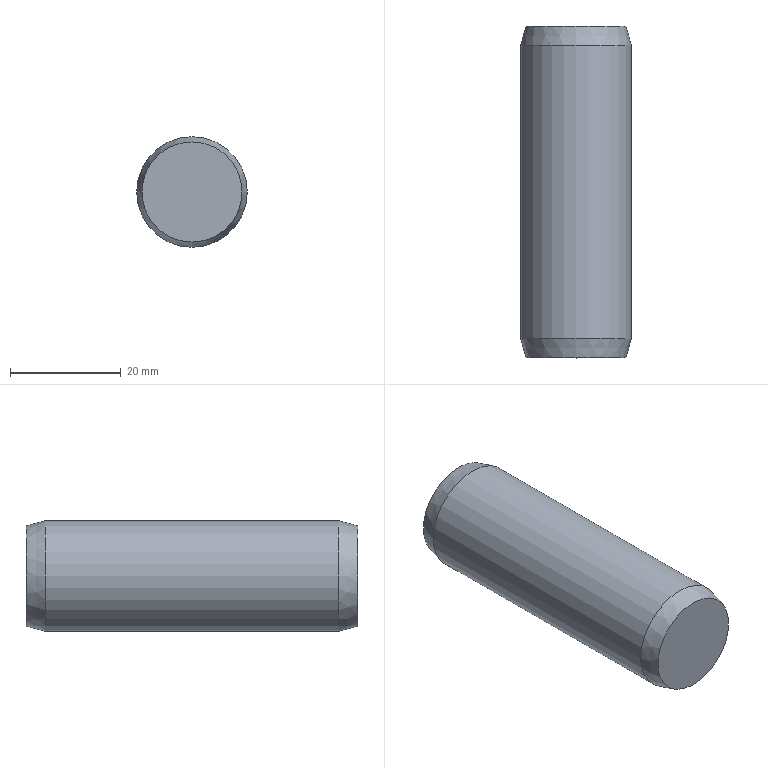Component | NX | GB-T119_1-2000_20X60 | 1 solid | 5 faces | box 20 x 60 x 20 mm | volume 18650 mm3 | plane 2 | cone 2 | cylinder 1 | commonest cylinder face diameters 20 x1
STEP:
#1=CARTESIAN_POINT('',(0.,0.,0.));
#2=DIRECTION('',(0.,0.,1.));
#3=DIRECTION('',(1.,0.,0.));
#4=AXIS2_PLACEMENT_3D('',#1,#2,#3);
#5=CARTESIAN_POINT('',(-170.,-110.,276.562));
#6=VERTEX_POINT('',#5);
#7=CARTESIAN_POINT('',(-170.,-110.,267.5));
#8=DIRECTION('',(0.,-1.,0.));
#9=DIRECTION('',(0.,0.,1.));
#10=AXIS2_PLACEMENT_3D('',#7,#8,#9);
#11=CIRCLE('',#10,9.062);
#12=CARTESIAN_POINT('',(-170.,-110.,267.5));
#13=DIRECTION('',(0.,-1.,0.));
#14=DIRECTION('',(0.,0.,1.));
#15=AXIS2_PLACEMENT_3D('',#12,#13,#14);
#16=PLANE('',#15);
#17=CARTESIAN_POINT('',(0.,0.));
#18=DIRECTION('',(1.,0.));
#19=AXIS2_PLACEMENT_2D('',#17,#18);
#20=CIRCLE('',#19,9.062);
#21=(GEOMETRIC_REPRESENTATION_CONTEXT(2)PARAMETRIC_REPRESENTATION_CONTEXT()REPRESENTATION_CONTEXT('',''));
#22=DEFINITIONAL_REPRESENTATION('',(#20),#21);
#23=PCURVE('',#16,#22);
#24=CARTESIAN_POINT('',(-170.,-110.,267.5));
#25=DIRECTION('',(0.,1.,0.));
#26=DIRECTION('',(0.,0.,-1.));
#27=AXIS2_PLACEMENT_3D('',#24,#25,#26);
#28=CONICAL_SURFACE('',#27,9.062,0.2618);
#29=CARTESIAN_POINT('',(9.425,-0.));
#30=DIRECTION('',(-1.,0.));
#31=VECTOR('',#30,1.);
#32=LINE('',#29,#31);
#33=(GEOMETRIC_REPRESENTATION_CONTEXT(2)PARAMETRIC_REPRESENTATION_CONTEXT()REPRESENTATION_CONTEXT('',''));
#34=DEFINITIONAL_REPRESENTATION('',(#32),#33);
#35=PCURVE('',#28,#34);
#36=SURFACE_CURVE('',#11,(#23,#35),.PCURVE_S1.);
#37=EDGE_CURVE('',#6,#6,#36,.T.);
#38=ORIENTED_EDGE('',*,*,#37,.T.);
#39=EDGE_LOOP('',(#38));
#40=FACE_BOUND('',#39,.T.);
#41=ADVANCED_FACE('',(#40),#16,.T.);
#42=CARTESIAN_POINT('',(-170.,-106.5,277.5));
#43=VERTEX_POINT('',#42);
#44=CARTESIAN_POINT('',(-170.,-106.5,267.5));
#45=DIRECTION('',(0.,-1.,0.));
#46=DIRECTION('',(0.,0.,1.));
#47=AXIS2_PLACEMENT_3D('',#44,#45,#46);
#48=CIRCLE('',#47,10.);
#49=CARTESIAN_POINT('',(9.425,3.5));
#50=DIRECTION('',(-1.,0.));
#51=VECTOR('',#50,1.);
#52=LINE('',#49,#51);
#53=(GEOMETRIC_REPRESENTATION_CONTEXT(2)PARAMETRIC_REPRESENTATION_CONTEXT()REPRESENTATION_CONTEXT('',''));
#54=DEFINITIONAL_REPRESENTATION('',(#52),#53);
#55=PCURVE('',#28,#54);
#56=CARTESIAN_POINT('',(-170.,-50.,267.5));
#57=DIRECTION('',(0.,-1.,0.));
#58=DIRECTION('',(0.,0.,1.));
#59=AXIS2_PLACEMENT_3D('',#56,#57,#58);
#60=CYLINDRICAL_SURFACE('',#59,10.);
#61=CARTESIAN_POINT('',(0.,56.5));
#62=DIRECTION('',(1.,0.));
#63=VECTOR('',#62,1.);
#64=LINE('',#61,#63);
#65=(GEOMETRIC_REPRESENTATION_CONTEXT(2)PARAMETRIC_REPRESENTATION_CONTEXT()REPRESENTATION_CONTEXT('',''));
#66=DEFINITIONAL_REPRESENTATION('',(#64),#65);
#67=PCURVE('',#60,#66);
#68=SURFACE_CURVE('',#48,(#55,#67),.PCURVE_S1.);
#69=EDGE_CURVE('',#43,#43,#68,.T.);
#70=ORIENTED_EDGE('',*,*,#69,.T.);
#71=CARTESIAN_POINT('',(-170.,-110.,276.562));
#72=CARTESIAN_POINT('',(-170.,-106.5,277.5));
#73=B_SPLINE_CURVE_WITH_KNOTS('',1,(#71,#72),.UNSPECIFIED.,.F.,.F.,(2,2),(-0.,3.623),.PIECEWISE_BEZIER_KNOTS.);
#74=CARTESIAN_POINT('',(3.142,0.));
#75=DIRECTION('',(0.,1.));
#76=VECTOR('',#75,1.);
#77=LINE('',#74,#76);
#78=(GEOMETRIC_REPRESENTATION_CONTEXT(2)PARAMETRIC_REPRESENTATION_CONTEXT()REPRESENTATION_CONTEXT('',''));
#79=DEFINITIONAL_REPRESENTATION('',(#77),#78);
#80=PCURVE('',#28,#79);
#81=CARTESIAN_POINT('',(9.425,0.));
#82=DIRECTION('',(0.,1.));
#83=VECTOR('',#82,1.);
#84=LINE('',#81,#83);
#85=(GEOMETRIC_REPRESENTATION_CONTEXT(2)PARAMETRIC_REPRESENTATION_CONTEXT()REPRESENTATION_CONTEXT('',''));
#86=DEFINITIONAL_REPRESENTATION('',(#84),#85);
#87=PCURVE('',#28,#86);
#88=SEAM_CURVE('',#73,(#80,#87),.PCURVE_S1.);
#89=EDGE_CURVE('',#6,#43,#88,.T.);
#90=ORIENTED_EDGE('',*,*,#89,.F.);
#91=ORIENTED_EDGE('',*,*,#37,.F.);
#92=ORIENTED_EDGE('',*,*,#89,.T.);
#93=EDGE_LOOP('',(#70,#90,#91,#92));
#94=FACE_BOUND('',#93,.T.);
#95=ADVANCED_FACE('',(#94),#28,.T.);
#96=CARTESIAN_POINT('',(-170.,-53.5,277.5));
#97=VERTEX_POINT('',#96);
#98=CARTESIAN_POINT('',(-170.,-53.5,267.5));
#99=DIRECTION('',(0.,-1.,0.));
#100=DIRECTION('',(0.,0.,1.));
#101=AXIS2_PLACEMENT_3D('',#98,#99,#100);
#102=CIRCLE('',#101,10.);
#103=CARTESIAN_POINT('',(0.,3.5));
#104=DIRECTION('',(1.,0.));
#105=VECTOR('',#104,1.);
#106=LINE('',#103,#105);
#107=(GEOMETRIC_REPRESENTATION_CONTEXT(2)PARAMETRIC_REPRESENTATION_CONTEXT()REPRESENTATION_CONTEXT('',''));
#108=DEFINITIONAL_REPRESENTATION('',(#106),#107);
#109=PCURVE('',#60,#108);
#110=CARTESIAN_POINT('',(-170.,-53.5,267.5));
#111=DIRECTION('',(0.,-1.,0.));
#112=DIRECTION('',(0.,0.,1.));
#113=AXIS2_PLACEMENT_3D('',#110,#111,#112);
#114=CONICAL_SURFACE('',#113,10.,0.2618);
#115=CARTESIAN_POINT('',(0.,0.));
#116=DIRECTION('',(1.,0.));
#117=VECTOR('',#116,1.);
#118=LINE('',#115,#117);
#119=(GEOMETRIC_REPRESENTATION_CONTEXT(2)PARAMETRIC_REPRESENTATION_CONTEXT()REPRESENTATION_CONTEXT('',''));
#120=DEFINITIONAL_REPRESENTATION('',(#118),#119);
#121=PCURVE('',#114,#120);
#122=SURFACE_CURVE('',#102,(#109,#121),.PCURVE_S1.);
#123=EDGE_CURVE('',#97,#97,#122,.T.);
#124=ORIENTED_EDGE('',*,*,#123,.T.);
#125=CARTESIAN_POINT('',(-170.,-53.5,277.5));
#126=CARTESIAN_POINT('',(-170.,-106.5,277.5));
#127=B_SPLINE_CURVE_WITH_KNOTS('',1,(#125,#126),.UNSPECIFIED.,.F.,.F.,(2,2),(3.5,56.5),.PIECEWISE_BEZIER_KNOTS.);
#128=CARTESIAN_POINT('',(6.283,0.));
#129=DIRECTION('',(0.,1.));
#130=VECTOR('',#129,1.);
#131=LINE('',#128,#130);
#132=(GEOMETRIC_REPRESENTATION_CONTEXT(2)PARAMETRIC_REPRESENTATION_CONTEXT()REPRESENTATION_CONTEXT('',''));
#133=DEFINITIONAL_REPRESENTATION('',(#131),#132);
#134=PCURVE('',#60,#133);
#135=CARTESIAN_POINT('',(0.,0.));
#136=DIRECTION('',(0.,1.));
#137=VECTOR('',#136,1.);
#138=LINE('',#135,#137);
#139=(GEOMETRIC_REPRESENTATION_CONTEXT(2)PARAMETRIC_REPRESENTATION_CONTEXT()REPRESENTATION_CONTEXT('',''));
#140=DEFINITIONAL_REPRESENTATION('',(#138),#139);
#141=PCURVE('',#60,#140);
#142=SEAM_CURVE('',#127,(#134,#141),.PCURVE_S1.);
#143=EDGE_CURVE('',#97,#43,#142,.T.);
#144=ORIENTED_EDGE('',*,*,#143,.T.);
#145=ORIENTED_EDGE('',*,*,#69,.F.);
#146=ORIENTED_EDGE('',*,*,#143,.F.);
#147=EDGE_LOOP('',(#124,#144,#145,#146));
#148=FACE_BOUND('',#147,.T.);
#149=ADVANCED_FACE('',(#148),#60,.T.);
#150=CARTESIAN_POINT('',(-170.,-50.,276.562));
#151=VERTEX_POINT('',#150);
#152=CARTESIAN_POINT('',(-170.,-50.,267.5));
#153=DIRECTION('',(0.,-1.,0.));
#154=DIRECTION('',(0.,0.,1.));
#155=AXIS2_PLACEMENT_3D('',#152,#153,#154);
#156=CIRCLE('',#155,9.062);
#157=CARTESIAN_POINT('',(0.,-3.5));
#158=DIRECTION('',(1.,0.));
#159=VECTOR('',#158,1.);
#160=LINE('',#157,#159);
#161=(GEOMETRIC_REPRESENTATION_CONTEXT(2)PARAMETRIC_REPRESENTATION_CONTEXT()REPRESENTATION_CONTEXT('',''));
#162=DEFINITIONAL_REPRESENTATION('',(#160),#161);
#163=PCURVE('',#114,#162);
#164=CARTESIAN_POINT('',(-170.,-50.,258.438));
#165=DIRECTION('',(0.,1.,0.));
#166=DIRECTION('',(0.,0.,-1.));
#167=AXIS2_PLACEMENT_3D('',#164,#165,#166);
#168=PLANE('',#167);
#169=CARTESIAN_POINT('',(-18.124,0.));
#170=CARTESIAN_POINT('',(-18.124,15.696));
#171=CARTESIAN_POINT('',(-4.531,7.848));
#172=CARTESIAN_POINT('',(9.062,0.));
#173=CARTESIAN_POINT('',(-4.531,-7.848));
#174=CARTESIAN_POINT('',(-18.124,-15.696));
#175=CARTESIAN_POINT('',(-18.124,0.));
#176=(BOUNDED_CURVE()B_SPLINE_CURVE(2,(#169,#170,#171,#172,#173,#174,#175),.UNSPECIFIED.,.T.,.F.)B_SPLINE_CURVE_WITH_KNOTS((1,2,2,2,2,1),(-2.094,0.,2.094,4.189,6.283,8.378),.UNSPECIFIED.)CURVE()GEOMETRIC_REPRESENTATION_ITEM()RATIONAL_B_SPLINE_CURVE((1.,0.5,1.,0.5,1.,0.5,1.))REPRESENTATION_ITEM(''));
#177=(GEOMETRIC_REPRESENTATION_CONTEXT(2)PARAMETRIC_REPRESENTATION_CONTEXT()REPRESENTATION_CONTEXT('',''));
#178=DEFINITIONAL_REPRESENTATION('',(#176),#177);
#179=PCURVE('',#168,#178);
#180=SURFACE_CURVE('',#156,(#163,#179),.PCURVE_S1.);
#181=EDGE_CURVE('',#151,#151,#180,.T.);
#182=ORIENTED_EDGE('',*,*,#181,.T.);
#183=CARTESIAN_POINT('',(-170.,-50.,276.562));
#184=CARTESIAN_POINT('',(-170.,-53.5,277.5));
#185=B_SPLINE_CURVE_WITH_KNOTS('',1,(#183,#184),.UNSPECIFIED.,.F.,.F.,(2,2),(-3.623,0.),.PIECEWISE_BEZIER_KNOTS.);
#186=CARTESIAN_POINT('',(6.283,0.));
#187=DIRECTION('',(0.,1.));
#188=VECTOR('',#187,1.);
#189=LINE('',#186,#188);
#190=(GEOMETRIC_REPRESENTATION_CONTEXT(2)PARAMETRIC_REPRESENTATION_CONTEXT()REPRESENTATION_CONTEXT('',''));
#191=DEFINITIONAL_REPRESENTATION('',(#189),#190);
#192=PCURVE('',#114,#191);
#193=CARTESIAN_POINT('',(0.,0.));
#194=DIRECTION('',(0.,1.));
#195=VECTOR('',#194,1.);
#196=LINE('',#193,#195);
#197=(GEOMETRIC_REPRESENTATION_CONTEXT(2)PARAMETRIC_REPRESENTATION_CONTEXT()REPRESENTATION_CONTEXT('',''));
#198=DEFINITIONAL_REPRESENTATION('',(#196),#197);
#199=PCURVE('',#114,#198);
#200=SEAM_CURVE('',#185,(#192,#199),.PCURVE_S1.);
#201=EDGE_CURVE('',#151,#97,#200,.T.);
#202=ORIENTED_EDGE('',*,*,#201,.T.);
#203=ORIENTED_EDGE('',*,*,#123,.F.);
#204=ORIENTED_EDGE('',*,*,#201,.F.);
#205=EDGE_LOOP('',(#182,#202,#203,#204));
#206=FACE_BOUND('',#205,.T.);
#207=ADVANCED_FACE('',(#206),#114,.T.);
#208=ORIENTED_EDGE('',*,*,#181,.F.);
#209=EDGE_LOOP('',(#208));
#210=FACE_BOUND('',#209,.T.);
#211=ADVANCED_FACE('',(#210),#168,.T.);
#212=CLOSED_SHELL('',(#41,#95,#149,#207,#211));
#213=MANIFOLD_SOLID_BREP('',#212);
#214=(LENGTH_UNIT()NAMED_UNIT(*)SI_UNIT(.MILLI.,.METRE.));
#215=UNCERTAINTY_MEASURE_WITH_UNIT(LENGTH_MEASURE(0.00001),#214,'','');
#216=(NAMED_UNIT(*)PLANE_ANGLE_UNIT()SI_UNIT($,.RADIAN.));
#217=(NAMED_UNIT(*)SI_UNIT($,.STERADIAN.)SOLID_ANGLE_UNIT());
#218=(GEOMETRIC_REPRESENTATION_CONTEXT(3)GLOBAL_UNCERTAINTY_ASSIGNED_CONTEXT((#215))GLOBAL_UNIT_ASSIGNED_CONTEXT((#214,#216,#217))REPRESENTATION_CONTEXT('',''));
#219=ADVANCED_BREP_SHAPE_REPRESENTATION('',(#4,#213),#218);